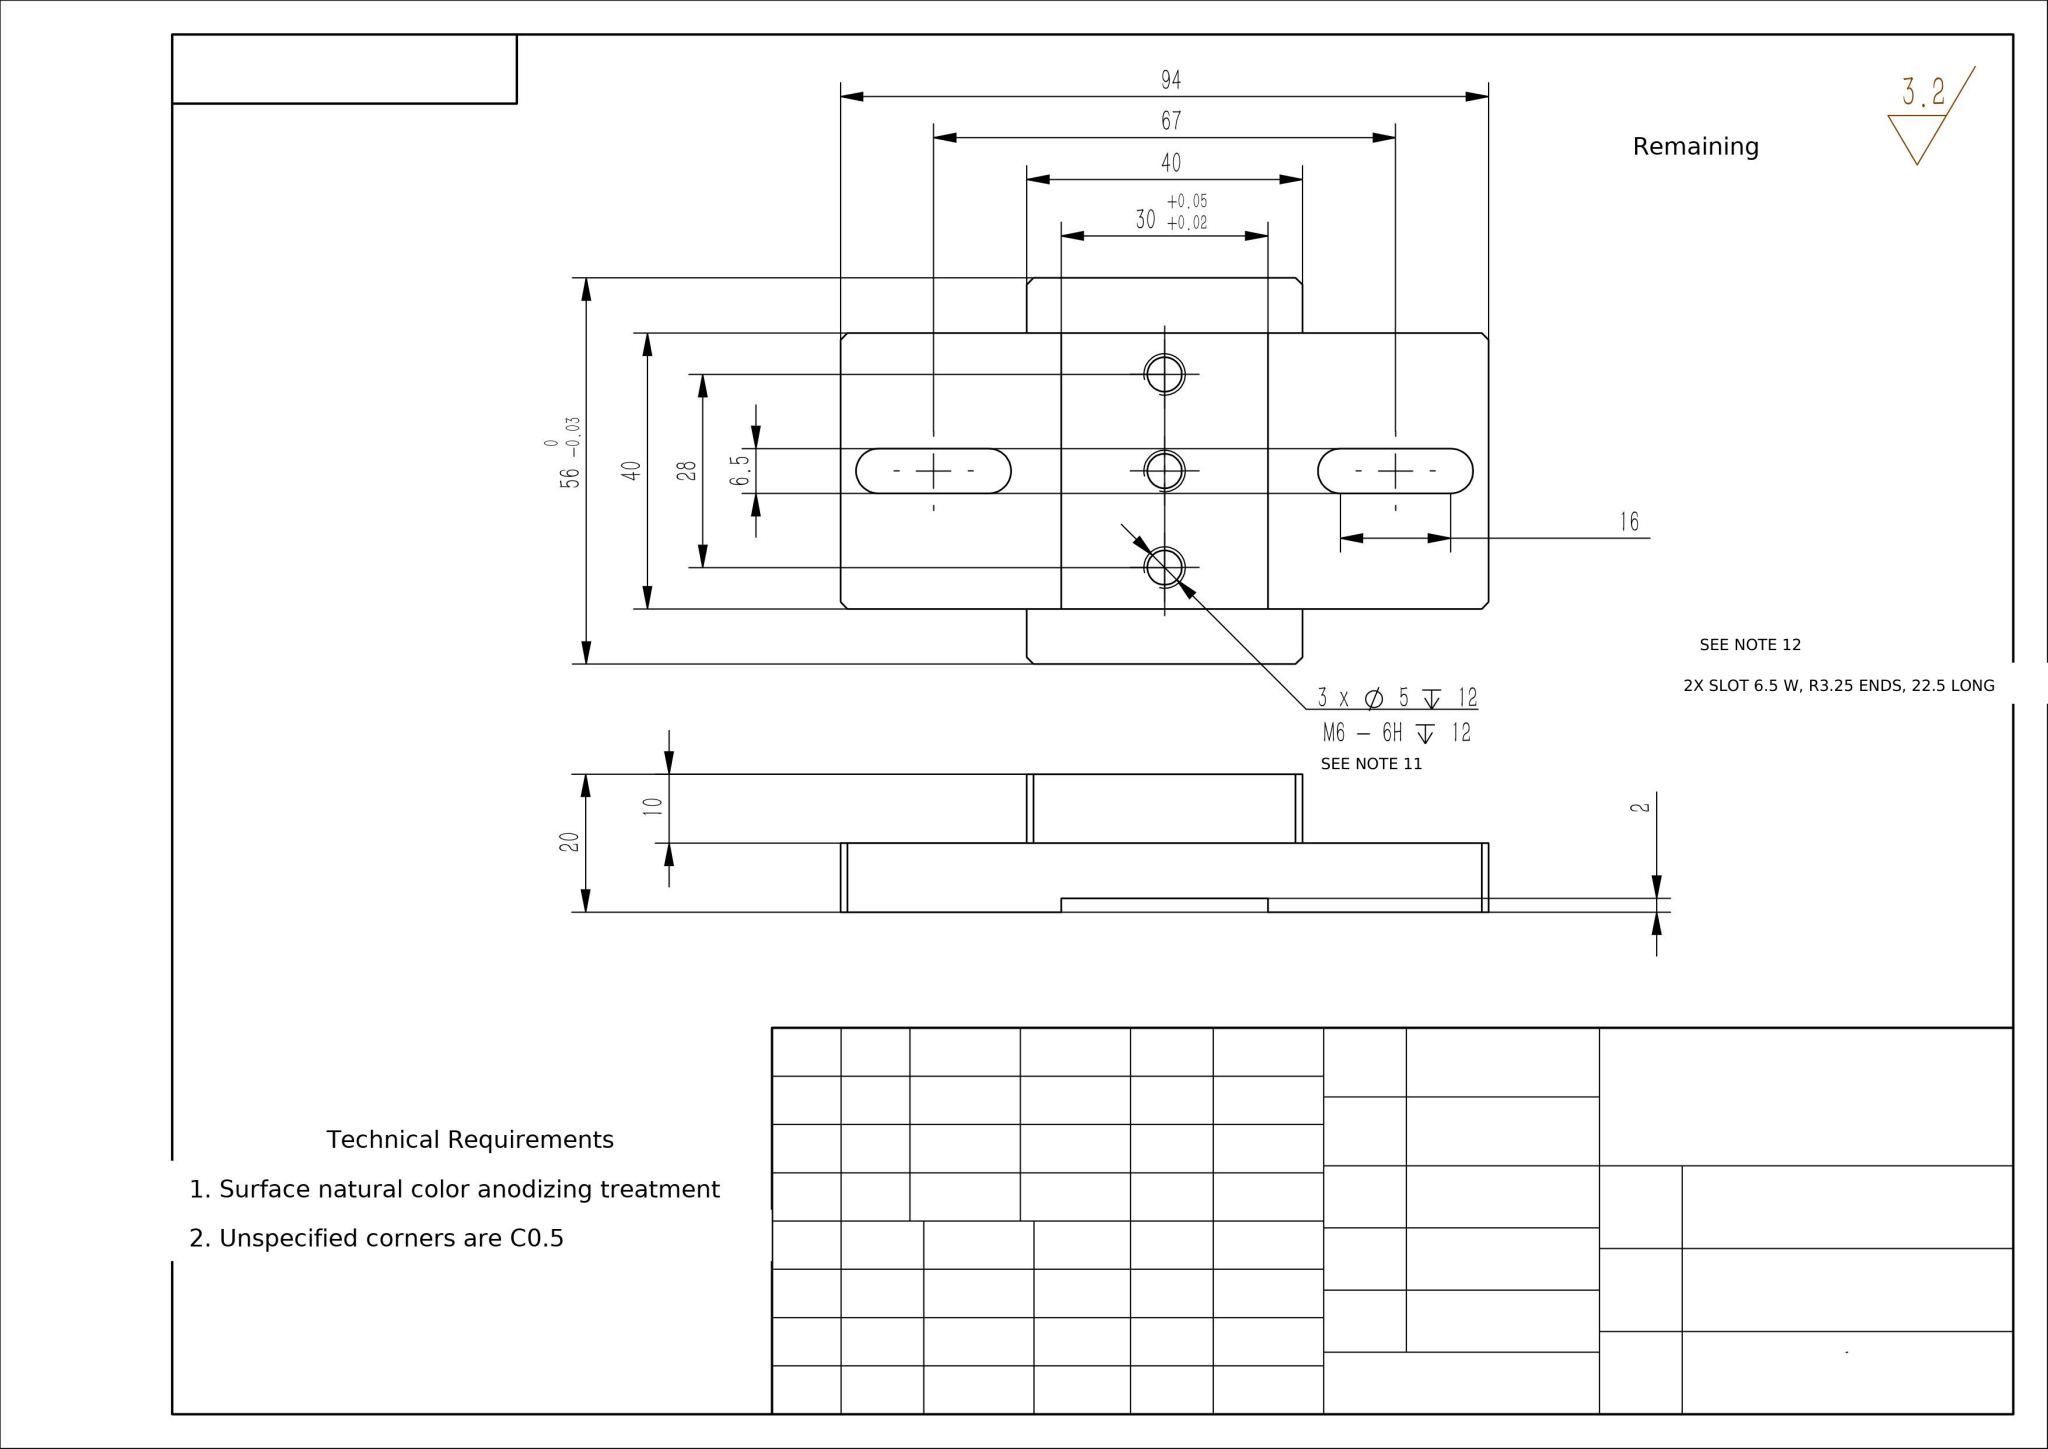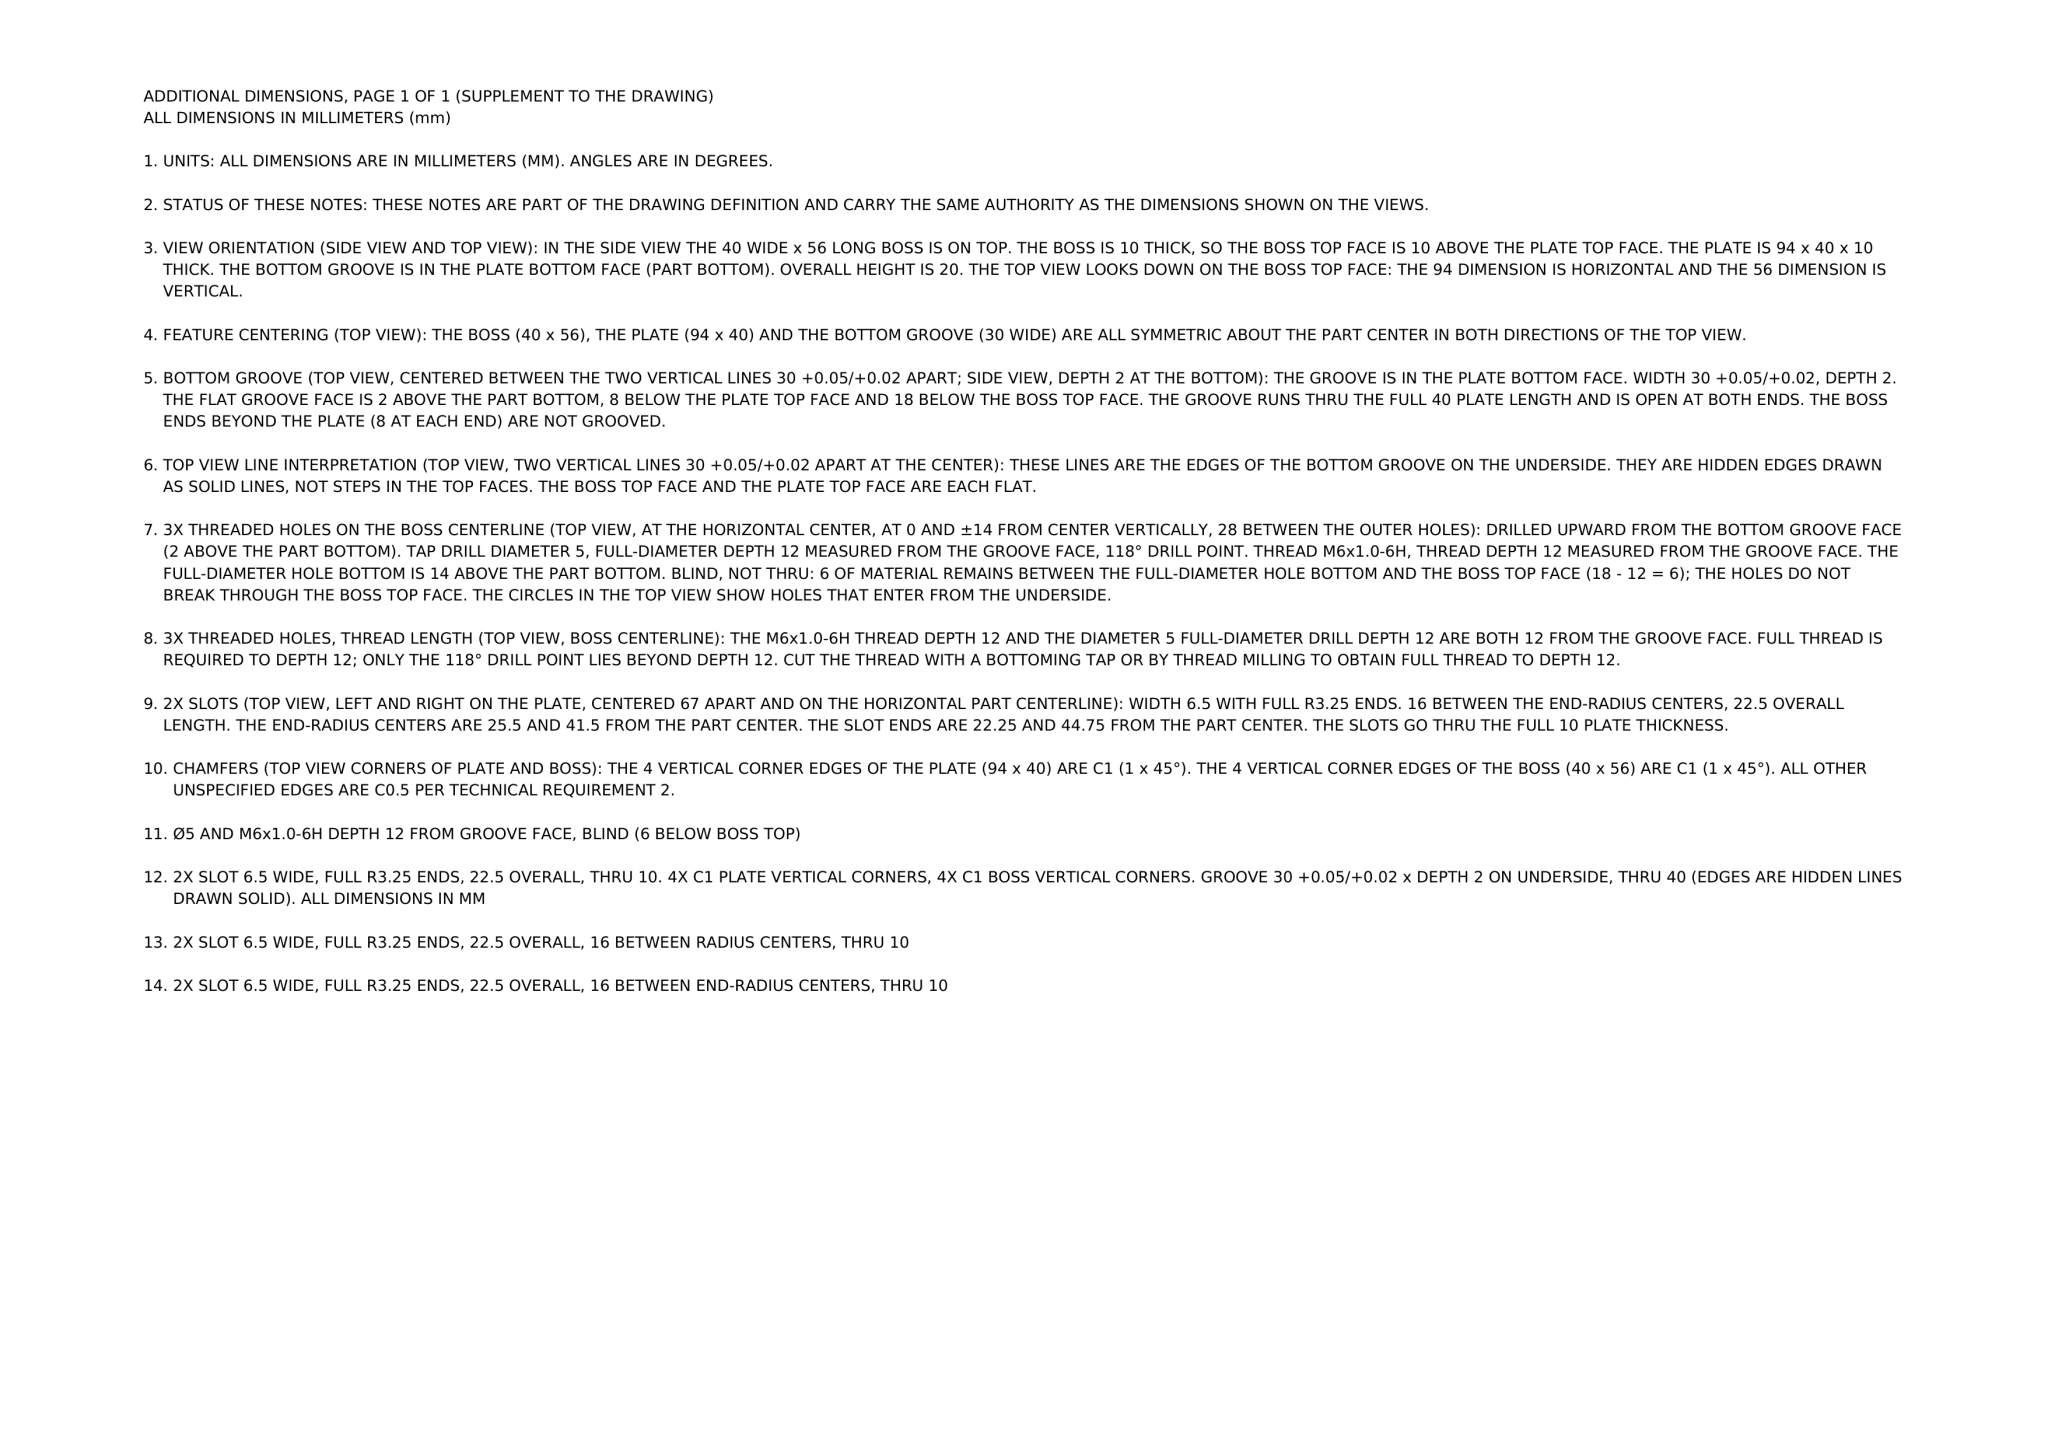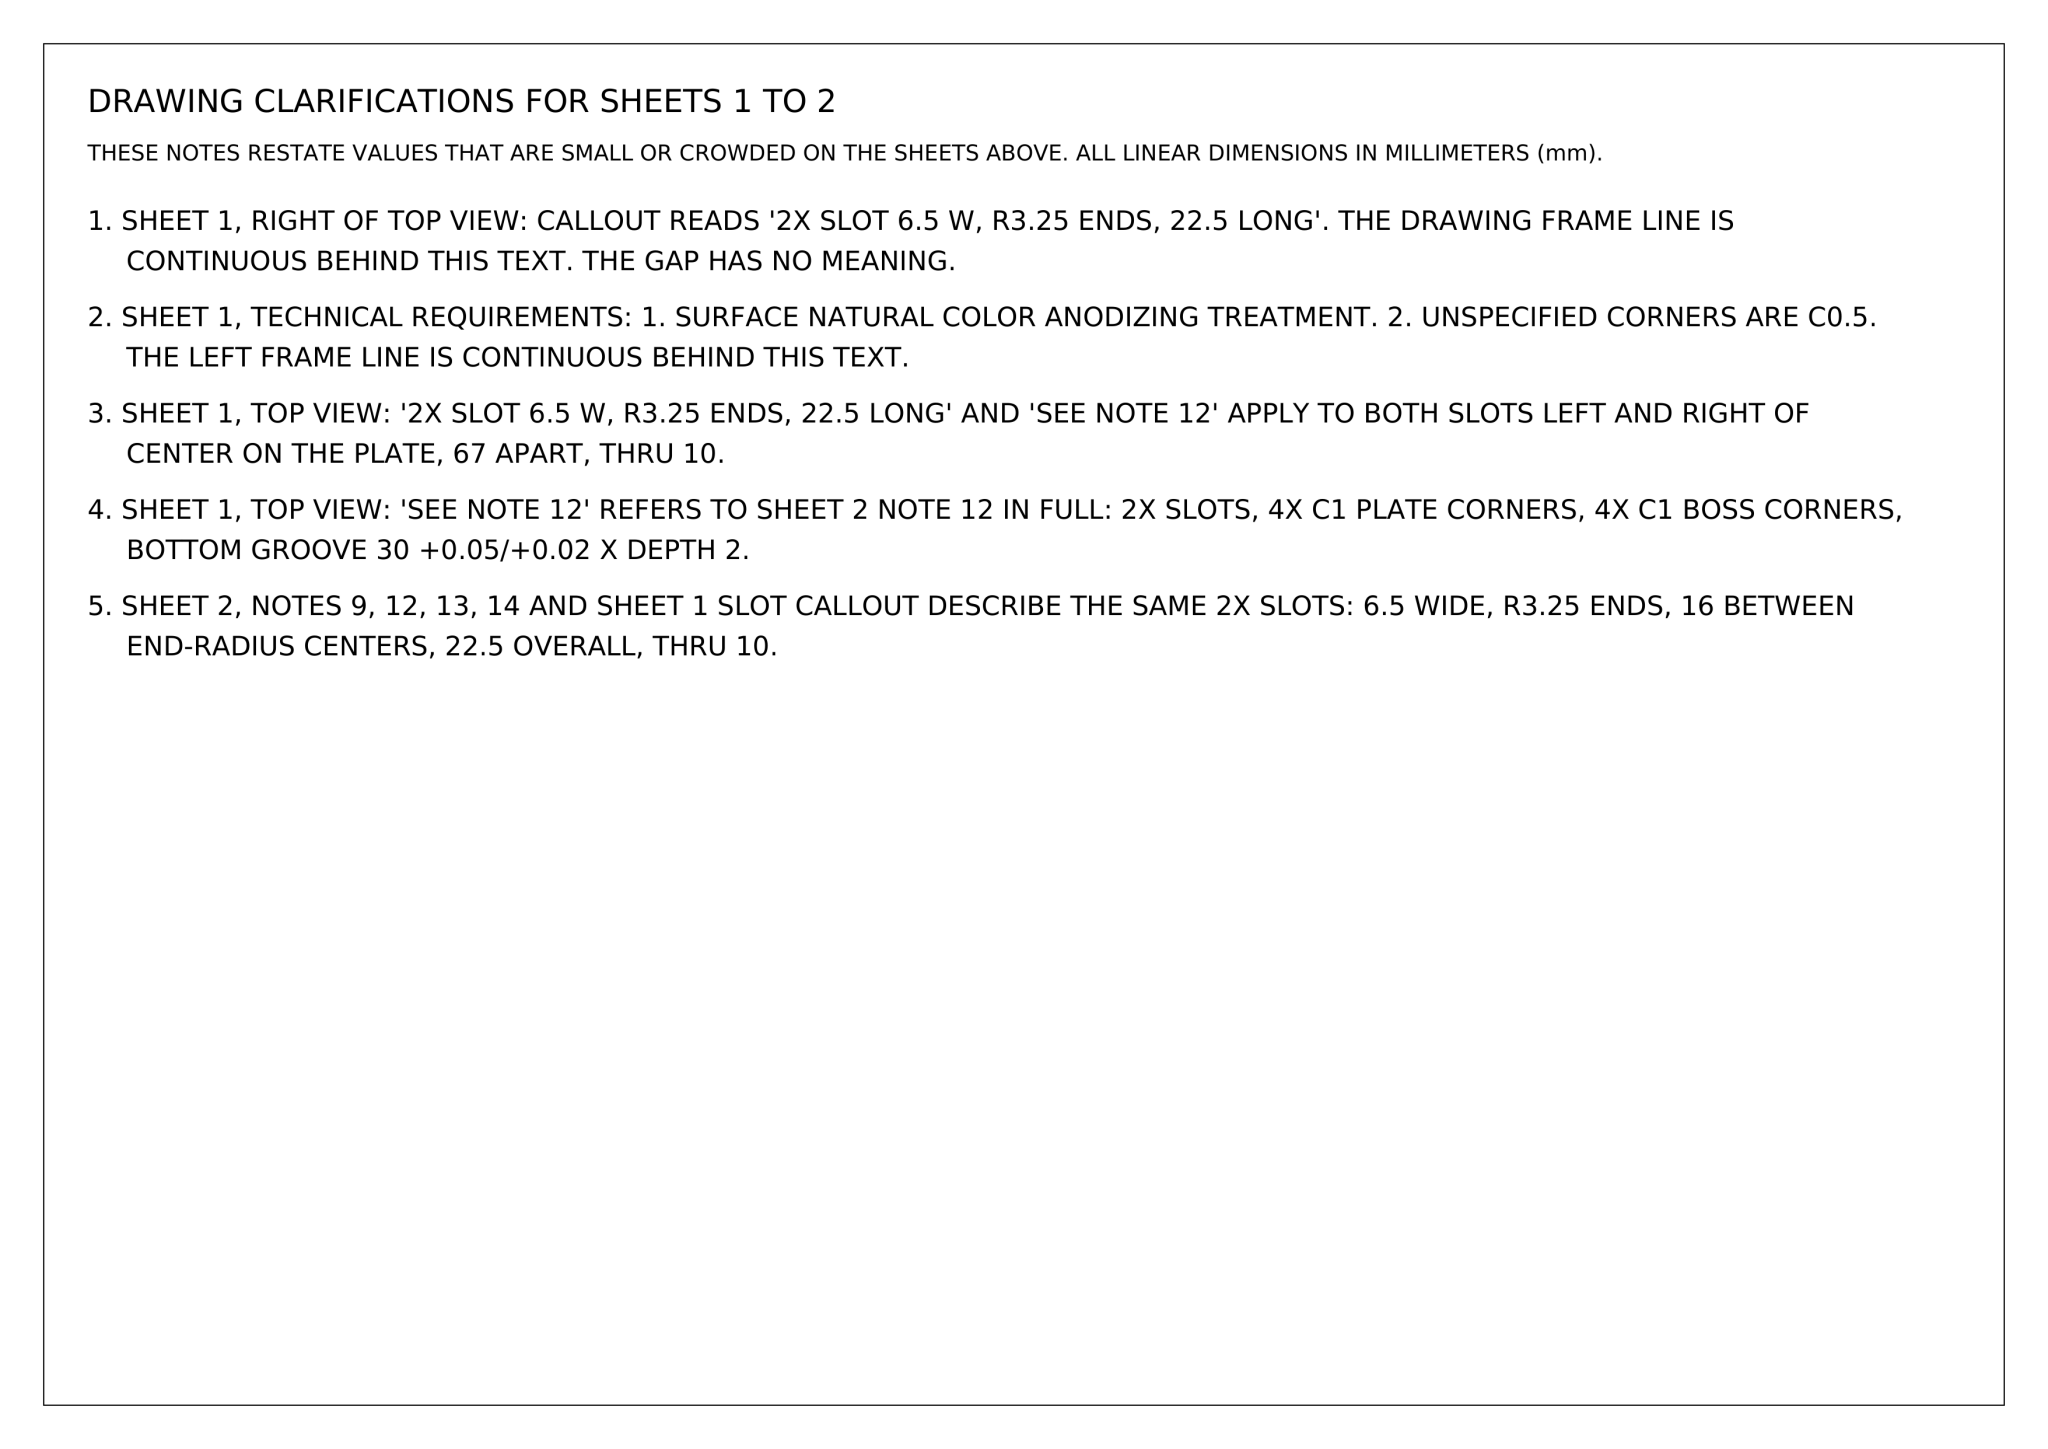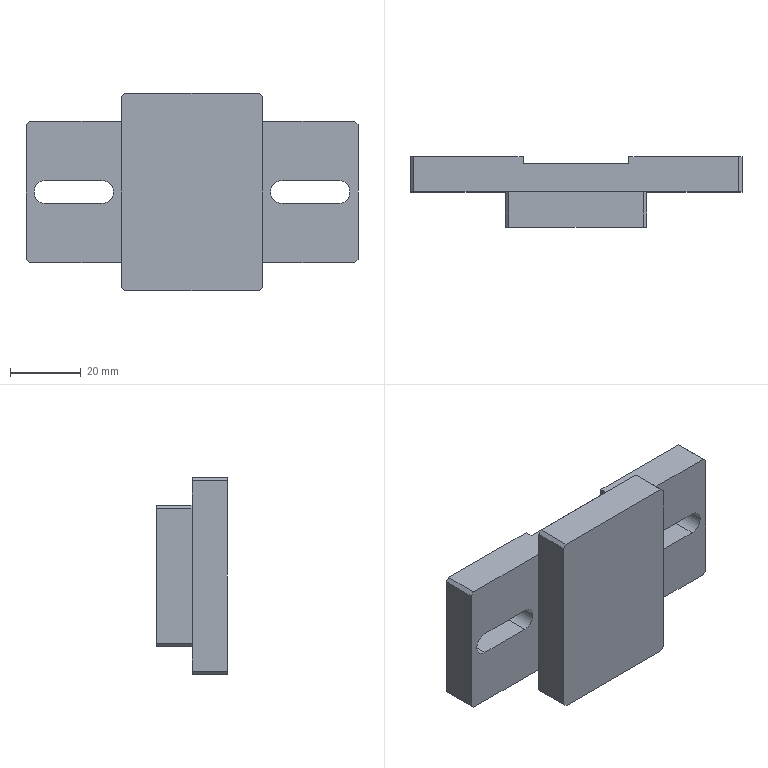Part | NX | mm | 1 solid | 46 faces | box 94 x 20 x 56 mm | volume 54080 mm3 | plane 30 | cylinder 10 | cone 6 | commonest cylinder face diameters 5 x6 6.5 x4